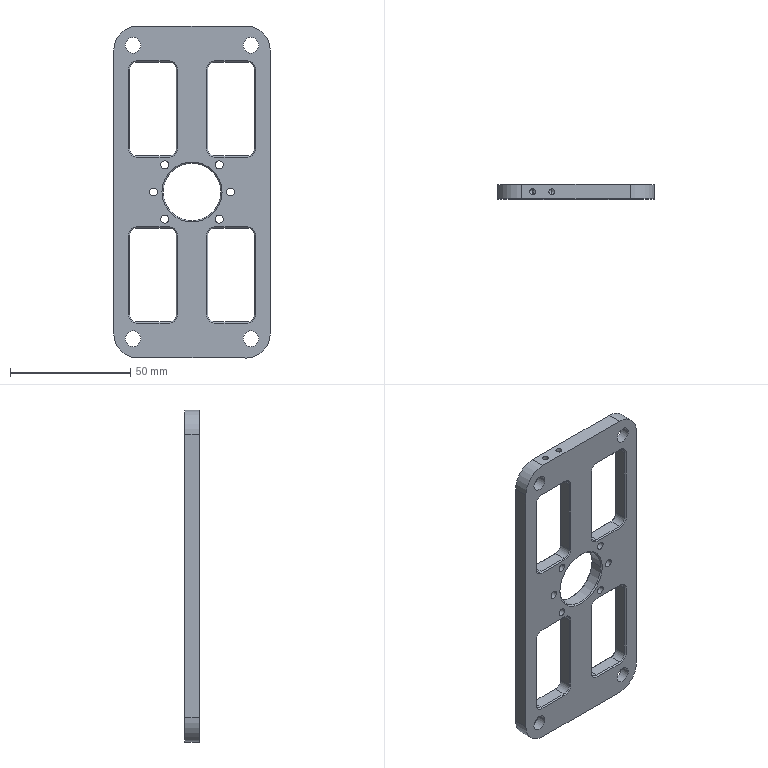Component | SolidWorks | F01AE00111-A2019-1 | 1 solid | 152 faces | box 65 x 6 x 138 mm | volume 30572 mm3 | plane 58 | cylinder 54 | cone 40 | commonest cylinder face diameters 6 x16 3.3 x12 12 x8 6.5 x8 2.5 x4 20 x4 24 x2
build123d program:
from build123d import *

# Parameters (mm, degrees)
SKETCH1_W             = 65
SKETCH1_H             = 138
SKETCH1_R             = 3.25
BOSS_EXTRUDE1_DEPTH   = 6
FILLET1_R             = 10
M3_TAPPED_HOLE1_D     = 2.5
M3_TAPPED_HOLE1_DEPTH = 7.5
M3_TAPPED_HOLE1_TIP   = 0.7511
CUT_EXTRUDE1_DEPTH    = 143.074
CHAMFER1_SIZE         = 0.5
SKETCH5_R             = 12
CUT_EXTRUDE2_DEPTH    = 143.074
M4_TAPPED_HOLE1_D     = 3.3
SKETCH8_R             = 6
CUT_EXTRUDE3_DEPTH    = 2
CHAMFER2_SIZE         = 0.5


with BuildPart() as part:
    # Sketch1 → Boss-Extrude1 (new body)
    with BuildSketch(Plane.XY):
        with Locations((24.5, -61)):
            Rectangle(SKETCH1_W, SKETCH1_H)
        with Locations((0, -122)):
            Circle(SKETCH1_R, mode=Mode.SUBTRACT)
        with Locations((49, -122)):
            Circle(SKETCH1_R, mode=Mode.SUBTRACT)
        Circle(SKETCH1_R, mode=Mode.SUBTRACT)
        with Locations((49, 0)):
            Circle(SKETCH1_R, mode=Mode.SUBTRACT)
    extrude(amount=BOSS_EXTRUDE1_DEPTH)

    # Fillet1
    fillet1_edges = [part.edges().sort_by_distance(p)[0] for p in [
        (-8, 8, 3),
        (57, 8, 3),
        (57, -130, 3),
        (-8, -130, 3),
    ]]
    fillet(fillet1_edges, radius=FILLET1_R)

    # M3 Tapped Hole1
    with Locations(Plane(origin=(0, 8, 0), x_dir=(1, 0, 0), z_dir=(0, 1, 0))):
        with Locations((6.5, -3), (14.5, -3)):
            Hole(M3_TAPPED_HOLE1_D / 2, depth=M3_TAPPED_HOLE1_DEPTH)
            with Locations((0, 0, -(M3_TAPPED_HOLE1_DEPTH + M3_TAPPED_HOLE1_TIP / 2))):  # 118° drill point
                Cone(0, M3_TAPPED_HOLE1_D / 2, M3_TAPPED_HOLE1_TIP, mode=Mode.SUBTRACT)

    # Sketch4 → Cut-Extrude1 (cut, through all)
    with BuildSketch(Plane(origin=(0, 0, 0), x_dir=(-1, 0, 0), z_dir=(0, 0, -1))):
        with BuildLine():
            Line((-18, -10), (-18, -43))
            ThreePointArc((-18, -43), (-17.121, -45.121), (-15, -46))
            Line((-15, -46), (-1.5, -46))
            ThreePointArc((-1.5, -46), (0.6213, -45.121), (1.5, -43))
            Line((1.5, -43), (1.5, -10))
            ThreePointArc((1.5, -10), (0.6213, -7.879), (-1.5, -7))
            Line((-1.5, -7), (-15, -7))
            ThreePointArc((-15, -7), (-17.121, -7.879), (-18, -10))
        make_face()
        with BuildLine():
            Line((-47.5, -7), (-34, -7))
            ThreePointArc((-34, -7), (-31.879, -7.879), (-31, -10))
            Line((-31, -10), (-31, -43))
            ThreePointArc((-31, -43), (-31.879, -45.121), (-34, -46))
            Line((-34, -46), (-47.5, -46))
            ThreePointArc((-47.5, -46), (-49.621, -45.121), (-50.5, -43))
            Line((-50.5, -43), (-50.5, -10))
            ThreePointArc((-50.5, -10), (-49.621, -7.879), (-47.5, -7))
        make_face()
        with BuildLine():
            Line((-1.5, -115), (-15, -115))
            ThreePointArc((-15, -115), (-17.121, -114.121), (-18, -112))
            Line((-18, -112), (-18, -79))
            ThreePointArc((-18, -79), (-17.121, -76.879), (-15, -76))
            Line((-15, -76), (-1.5, -76))
            ThreePointArc((-1.5, -76), (0.6213, -76.879), (1.5, -79))
            Line((1.5, -79), (1.5, -112))
            ThreePointArc((1.5, -112), (0.6213, -114.121), (-1.5, -115))
        make_face()
        with BuildLine():
            Line((-31, -112), (-31, -79))
            ThreePointArc((-31, -79), (-31.879, -76.879), (-34, -76))
            Line((-34, -76), (-47.5, -76))
            ThreePointArc((-47.5, -76), (-49.621, -76.879), (-50.5, -79))
            Line((-50.5, -79), (-50.5, -112))
            ThreePointArc((-50.5, -112), (-49.621, -114.121), (-47.5, -115))
            Line((-47.5, -115), (-34, -115))
            ThreePointArc((-34, -115), (-31.879, -114.121), (-31, -112))
        make_face()
    extrude(amount=-CUT_EXTRUDE1_DEPTH, mode=Mode.SUBTRACT)

    # Chamfer1
    chamfer1_edges = [part.edges().sort_by_distance(p)[0] for p in [
        (-1.5, -26.5, 0),
        (-0.6213, -76.879, 6),
        (-1.5, -95.5, 6),
        (-0.6213, -114.121, 6),
        (8.25, -115, 6),
        (17.121, -114.121, 6),
        (18, -95.5, 6),
        (17.121, -76.879, 6),
        (8.25, -76, 6),
        (-0.6213, -76.879, 0),
        (8.25, -76, 0),
        (17.121, -76.879, 0),
        (18, -95.5, 0),
        (17.121, -114.121, 0),
        (8.25, -115, 0),
        (-0.6213, -114.121, 0),
        (-1.5, -95.5, 0),
        (49.621, -114.121, 6),
        (50.5, -95.5, 6),
        (49.621, -76.879, 6),
        (40.75, -76, 6),
        (31.879, -76.879, 6),
        (31, -95.5, 6),
        (31.879, -114.121, 6),
        (40.75, -115, 6),
        (49.621, -114.121, 0),
        (40.75, -115, 0),
        (31.879, -114.121, 0),
        (31, -95.5, 0),
        (31.879, -76.879, 0),
        (40.75, -76, 0),
        (49.621, -76.879, 0),
        (50.5, -95.5, 0),
        (49.621, -45.121, 6),
        (50.5, -26.5, 6),
        (49.621, -7.879, 6),
        (40.75, -7, 6),
        (31.879, -7.879, 6),
        (31, -26.5, 6),
        (31.879, -45.121, 6),
        (40.75, -46, 6),
        (49.621, -45.121, 0),
        (40.75, -46, 0),
        (31.879, -45.121, 0),
        (31, -26.5, 0),
        (31.879, -7.879, 0),
        (40.75, -7, 0),
        (49.621, -7.879, 0),
        (50.5, -26.5, 0),
        (-0.6213, -7.879, 6),
        (-1.5, -26.5, 6),
        (-0.6213, -45.121, 6),
        (8.25, -46, 6),
        (17.121, -45.121, 6),
        (18, -26.5, 6),
        (17.121, -7.879, 6),
        (8.25, -7, 6),
        (-0.6213, -7.879, 0),
        (8.25, -7, 0),
        (17.121, -7.879, 0),
        (18, -26.5, 0),
        (17.121, -45.121, 0),
        (8.25, -46, 0),
        (-0.6213, -45.121, 0),
    ]]
    chamfer(chamfer1_edges, length=CHAMFER1_SIZE)

    # Sketch5 → Cut-Extrude2 (cut, through all)
    with BuildSketch(Plane(origin=(0, 0, 0), x_dir=(-1, 0, 0), z_dir=(0, 0, -1))):
        with Locations((-24.5, -61)):
            Circle(SKETCH5_R)
    extrude(amount=-CUT_EXTRUDE2_DEPTH, mode=Mode.SUBTRACT)

    # M4 Tapped Hole1 (through all)
    with Locations(Plane(origin=(0, 0, 0), x_dir=(-1, 0, 0), z_dir=(0, 0, -1))):
        with Locations((-35.814, -49.686), (-40.5, -61), (-35.814, -72.314), (-13.186, -72.314), (-8.5, -61), (-13.186, -49.686)):
            Hole(M4_TAPPED_HOLE1_D / 2)

    # Sketch8 → Cut-Extrude3 (cut)
    with BuildSketch(Plane(origin=(0, 0, 0), x_dir=(-1, 0, 0), z_dir=(0, 0, -1))):
        with Locations((-49, 0)):
            Circle(SKETCH8_R)
        Circle(SKETCH8_R)
        with Locations((-49, -122)):
            Circle(SKETCH8_R)
        with Locations((0, -122)):
            Circle(SKETCH8_R)
    extrude(amount=-CUT_EXTRUDE3_DEPTH, mode=Mode.SUBTRACT)

    # Chamfer2
    chamfer2_edges = [part.edges().sort_by_distance(p)[0] for p in [
        (36.5, -61, 6),
        (36.5, -61, 0),
    ]]
    chamfer(chamfer2_edges, length=CHAMFER2_SIZE)


solid = part.part

# Placed as in the assembly
solid = solid.moved(Location((-133.852, -190.452, -211.475), (90, 0, 0)))